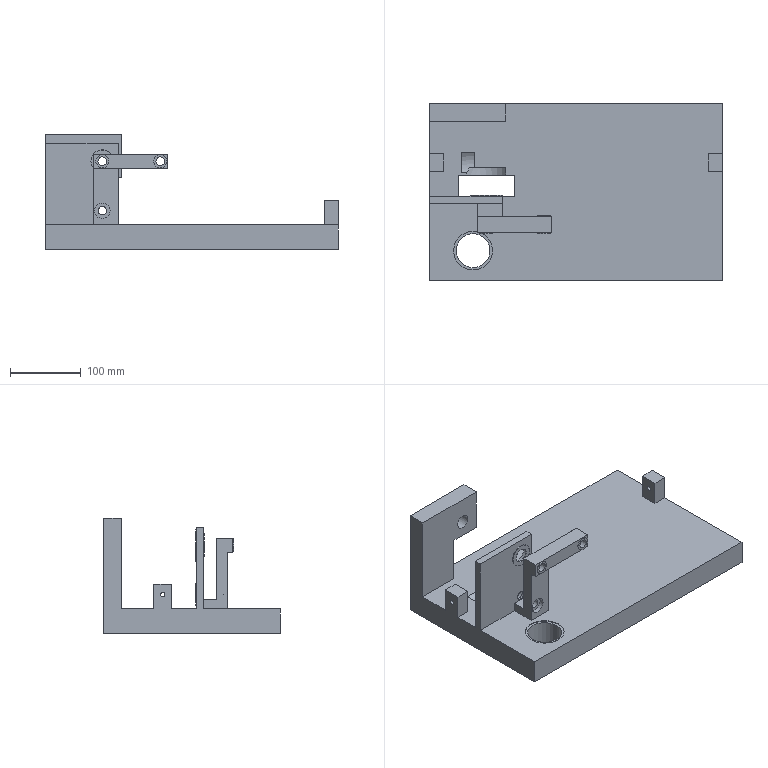Component | NX | BASE | 1 solid | 74 faces | volume 3957870 mm3 | plane 50 | cylinder 24 | commonest cylinder face diameters 18.5 x3 12 x2 20 x2 12.5 x2 37 x2 32 x2 22 x2 6 x2